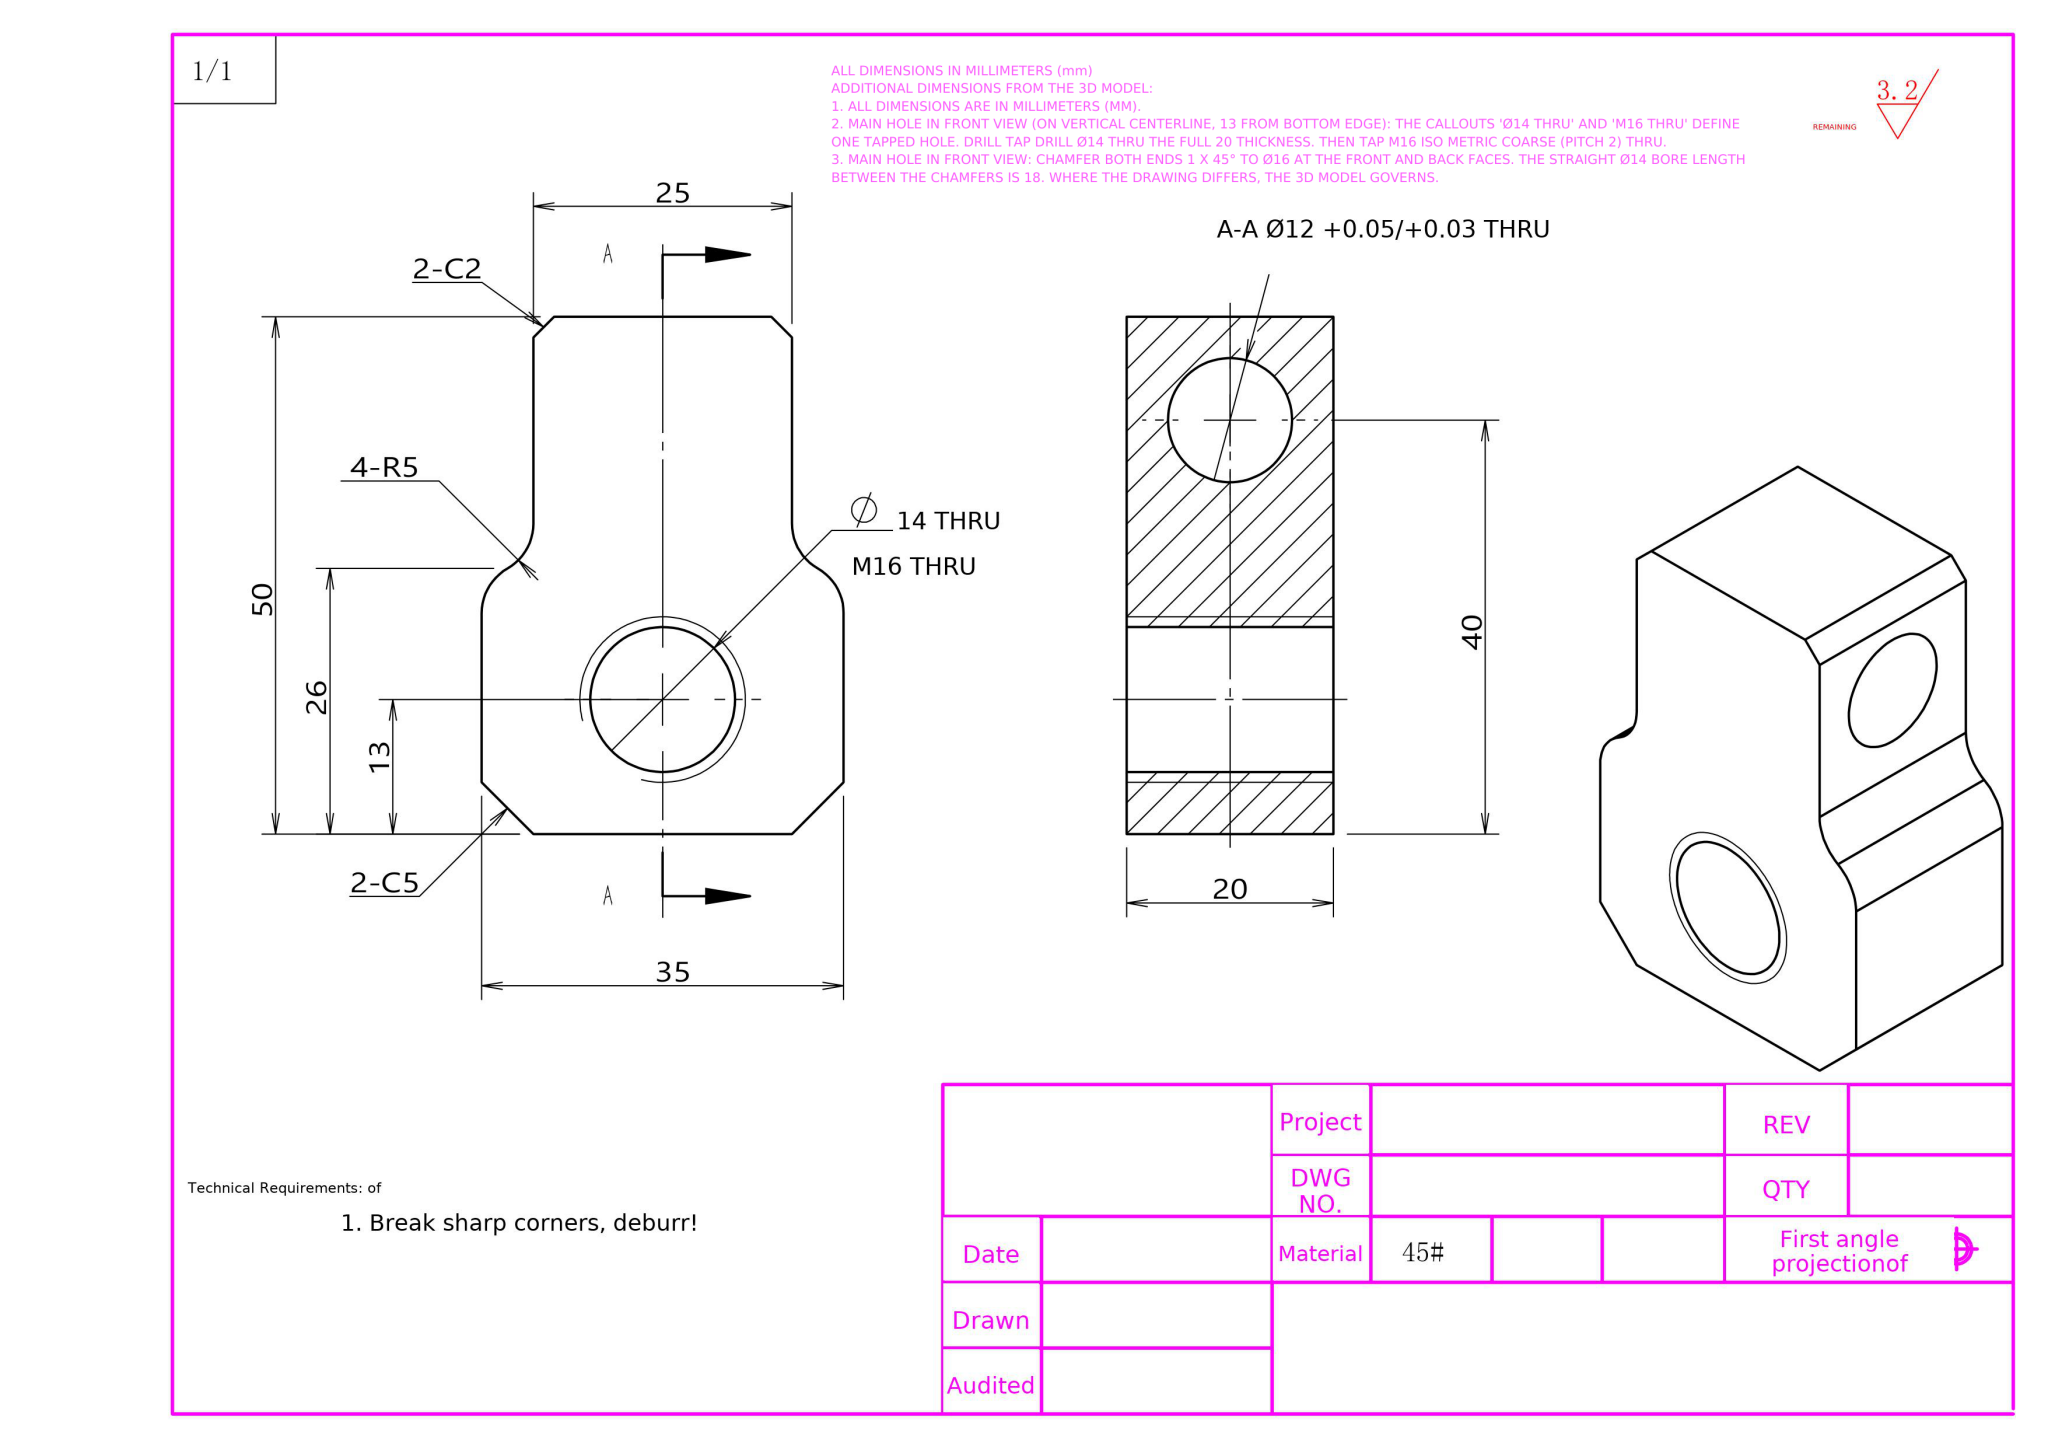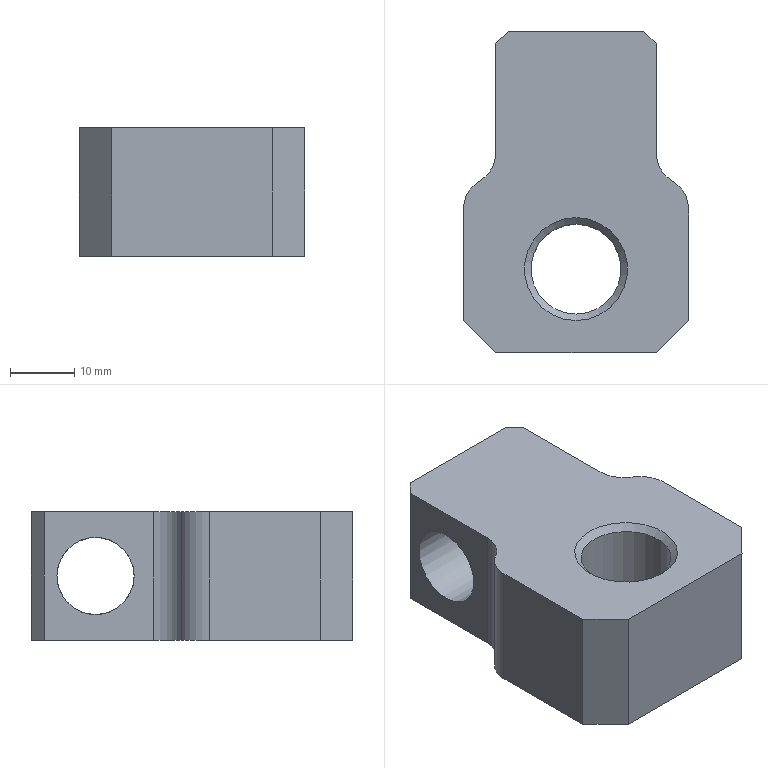Part | NX | mm | Shouldered Perpendicular Bore Block | 1 solid | 20 faces | box 35.01 x 50 x 20.01 mm | volume 23802 mm3 | plane 12 | cylinder 6 | cone 2 | commonest cylinder face diameters 10 x4 14 x1 12 x1